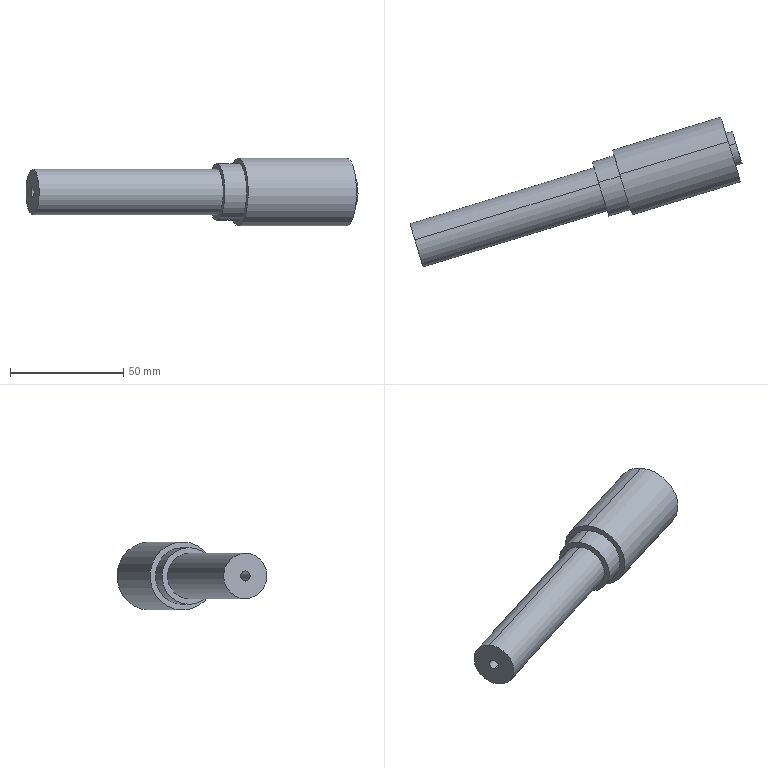Component | SolidWorks | V1ZHXTRotatingAxisSB1-1 | 1 solid | 34 faces | box 146.66 x 66.23 x 30 mm | volume 66443 mm3 | cylinder 20 | cone 8 | plane 6 | commonest cylinder face diameters 3.3 x6 4 x2 4.496 x2 15 x2 2 x2 30 x2 25 x2 20 x2
build123d program:
from build123d import *

# Parameters (mm, degrees)
SKETCH1_R                  = 10
BOSS_EXTRUDE1_DEPTH        = 85
SKETCH2_R                  = 12.5
BOSS_EXTRUDE2_DEPTH        = 10
SKETCH3_R                  = 15
BOSS_EXTRUDE3_DEPTH        = 50
SKETCH4_R                  = 1
CUT_EXTRUDE1_DEPTH         = 147.544
BOSS_EXTRUDE4_START        = 3
SKETCH5_R                  = 7.5
SKETCH5_R_2                = 1
BOSS_EXTRUDE4_DEPTH        = 3
M4_TAPPED_HOLE1_D          = 3.3
M4_TAPPED_HOLE1_DEPTH      = 10.1
M4_TAPPED_HOLE1_TIP        = 0.9914
F_12_24_TAPPED_HOLE1_D     = 4.496
F_12_24_TAPPED_HOLE1_DEPTH = 14.15
F_12_24_TAPPED_HOLE1_TIP   = 1.351
SKETCH10_R                 = 2
CUT_EXTRUDE2_DEPTH         = 10


with BuildPart() as part:
    # Sketch1 → Boss-Extrude1 (new body)
    with BuildSketch(Plane(origin=(0, 0, 0), x_dir=(1, 0, 0), z_dir=(0, 1, 0))):
        with Locations(Location((0, 0, 0), (0, 0, 270))):
            Circle(SKETCH1_R)
    extrude(amount=BOSS_EXTRUDE1_DEPTH)

    # Sketch2 → Boss-Extrude2 (add)
    with BuildSketch(Plane(origin=(0, 85, 0), x_dir=(1, 0, 0), z_dir=(0, 1, 0))):
        with Locations(Location((0, 0, 0), (0, 0, 270))):
            Circle(SKETCH2_R)
    extrude(amount=BOSS_EXTRUDE2_DEPTH)

    # Sketch3 → Boss-Extrude3 (add)
    with BuildSketch(Plane(origin=(0, 95, 0), x_dir=(1, 0, 0), z_dir=(0, 1, 0))):
        with Locations(Location((0, 0, 0), (0, 0, 270))):
            Circle(SKETCH3_R)
    extrude(amount=BOSS_EXTRUDE3_DEPTH)

    # Sketch4 → Cut-Extrude1 (cut, through all)
    with BuildSketch(Plane(origin=(0, 145, 0), x_dir=(1, 0, 0), z_dir=(0, 1, 0))):
        with Locations(Location((0, 0, 0), (0, 0, 270))):
            Circle(SKETCH4_R)
    extrude(amount=-CUT_EXTRUDE1_DEPTH, mode=Mode.SUBTRACT)

    # Sketch5 → Boss-Extrude4 (add)
    with BuildSketch(Plane(origin=(0, 145, 0), x_dir=(1, 0, 0), z_dir=(0, 1, 0)).offset(BOSS_EXTRUDE4_START)):
        with Locations(Location((0, 0, 0), (0, 0, 270))):
            Circle(SKETCH5_R)
        with Locations(Location((0, 0, 0), (0, 0, 270))):
            Circle(SKETCH5_R_2, mode=Mode.SUBTRACT)
    extrude(amount=-BOSS_EXTRUDE4_DEPTH)

    # M4 Tapped Hole1
    with Locations(Plane(origin=(0, 145, 0), x_dir=(1, 0, 0), z_dir=(0, 1, 0))):
        with Locations((0, 11), (-9.526, -5.5), (9.526, -5.5)):
            Hole(M4_TAPPED_HOLE1_D / 2, depth=M4_TAPPED_HOLE1_DEPTH)
            with Locations((0, 0, -(M4_TAPPED_HOLE1_DEPTH + M4_TAPPED_HOLE1_TIP / 2))):  # 118° drill point
                Cone(0, M4_TAPPED_HOLE1_D / 2, M4_TAPPED_HOLE1_TIP, mode=Mode.SUBTRACT)

    # 12-24 Tapped Hole1
    with Locations(Plane(origin=(0, 0, 0), x_dir=(-1, 0, 0), z_dir=(0, -1, 0))):
        with Locations((0, 0)):
            Hole(F_12_24_TAPPED_HOLE1_D / 2, depth=F_12_24_TAPPED_HOLE1_DEPTH)
            with Locations((0, 0, -(F_12_24_TAPPED_HOLE1_DEPTH + F_12_24_TAPPED_HOLE1_TIP / 2))):  # 118° drill point
                Cone(0, F_12_24_TAPPED_HOLE1_D / 2, F_12_24_TAPPED_HOLE1_TIP, mode=Mode.SUBTRACT)

    # Sketch10 → Cut-Extrude2 (cut)
    with BuildSketch(Plane(origin=(0, 145, 0), x_dir=(1, 0, 0), z_dir=(0, 1, 0))):
        with Locations(Location((9.526, 5.5, 0), (0, 0, 270))):
            Circle(SKETCH10_R)
    extrude(amount=-CUT_EXTRUDE2_DEPTH, mode=Mode.SUBTRACT)


solid = part.part

# Placed as in the assembly
solid = solid.moved(Location((147.067, -241.347, 375.239), (-13.538, -4.085, -73.517)))
STEP:
#1=COLOUR_RGB('',0.7922,0.8196,0.9333);
#2=FILL_AREA_STYLE_COLOUR('',#1);
#3=FILL_AREA_STYLE('',(#2));
#4=SURFACE_STYLE_FILL_AREA(#3);
#5=SURFACE_SIDE_STYLE('',(#4));
#6=SURFACE_STYLE_USAGE(.BOTH.,#5);
#7=PRESENTATION_STYLE_ASSIGNMENT((#6));
#8=CARTESIAN_POINT('',(11.001,-8.368,14.578));
#9=VERTEX_POINT('',#8);
#10=CARTESIAN_POINT('',(10.99,-8.331,14.731));
#11=VERTEX_POINT('',#10);
#12=CARTESIAN_POINT('',(10.995,-8.349,14.655));
#13=DIRECTION('',(0.9565,0.2918,0.));
#14=DIRECTION('',(-0.07124,0.2335,0.9697));
#15=AXIS2_PLACEMENT_3D('',#12,#13,#14);
#16=CIRCLE('',#15,0.07874);
#17=EDGE_CURVE('',#9,#11,#16,.T.);
#18=ORIENTED_EDGE('',*,*,#17,.F.);
#19=CARTESIAN_POINT('',(11.377,-8.253,14.578));
#20=VERTEX_POINT('',#19);
#21=CARTESIAN_POINT('',(11.001,-8.368,14.578));
#22=DIRECTION('',(0.9565,0.2918,0.));
#23=VECTOR('',#22,39.37);
#24=LINE('',#21,#23);
#25=EDGE_CURVE('',#9,#20,#24,.T.);
#26=ORIENTED_EDGE('',*,*,#25,.T.);
#27=CARTESIAN_POINT('',(11.366,-8.216,14.731));
#28=VERTEX_POINT('',#27);
#29=CARTESIAN_POINT('',(11.372,-8.234,14.655));
#30=DIRECTION('',(0.9565,0.2918,0.));
#31=DIRECTION('',(-0.07124,0.2335,0.9697));
#32=AXIS2_PLACEMENT_3D('',#29,#30,#31);
#33=CIRCLE('',#32,0.07874);
#34=EDGE_CURVE('',#20,#28,#33,.T.);
#35=ORIENTED_EDGE('',*,*,#34,.T.);
#36=CARTESIAN_POINT('',(10.99,-8.331,14.731));
#37=DIRECTION('',(0.9565,0.2918,0.));
#38=VECTOR('',#37,39.37);
#39=LINE('',#36,#38);
#40=EDGE_CURVE('',#11,#28,#39,.T.);
#41=ORIENTED_EDGE('',*,*,#40,.F.);
#42=EDGE_LOOP('',(#18,#26,#35,#41));
#43=FACE_OUTER_BOUND('',#42,.T.);
#44=CARTESIAN_POINT('',(10.995,-8.349,14.655));
#45=DIRECTION('',(0.9565,0.2918,0.));
#46=DIRECTION('',(-0.07124,0.2335,0.9697));
#47=AXIS2_PLACEMENT_3D('',#44,#45,#46);
#48=CYLINDRICAL_SURFACE('',#47,0.07874);
#49=ADVANCED_FACE('',(#43),#48,.F.);
#50=CARTESIAN_POINT('',(6.317,-9.319,14.859));
#51=VERTEX_POINT('',#50);
#52=CARTESIAN_POINT('',(6.329,-9.36,14.687));
#53=VERTEX_POINT('',#52);
#54=CARTESIAN_POINT('',(6.323,-9.339,14.773));
#55=DIRECTION('',(-0.9565,-0.2918,-0.));
#56=DIRECTION('',(0.07124,-0.2335,-0.9697));
#57=AXIS2_PLACEMENT_3D('',#54,#55,#56);
#58=CIRCLE('',#57,0.0885);
#59=EDGE_CURVE('',#51,#53,#58,.T.);
#60=ORIENTED_EDGE('',*,*,#59,.F.);
#61=CARTESIAN_POINT('',(5.784,-9.481,14.859));
#62=VERTEX_POINT('',#61);
#63=CARTESIAN_POINT('',(5.784,-9.481,14.859));
#64=DIRECTION('',(-0.9565,-0.2918,-0.));
#65=VECTOR('',#64,39.37);
#66=LINE('',#63,#65);
#67=EDGE_CURVE('',#51,#62,#66,.T.);
#68=ORIENTED_EDGE('',*,*,#67,.T.);
#69=CARTESIAN_POINT('',(5.796,-9.523,14.687));
#70=VERTEX_POINT('',#69);
#71=CARTESIAN_POINT('',(5.79,-9.502,14.773));
#72=DIRECTION('',(-0.9565,-0.2918,-0.));
#73=DIRECTION('',(0.07124,-0.2335,-0.9697));
#74=AXIS2_PLACEMENT_3D('',#71,#72,#73);
#75=CIRCLE('',#74,0.0885);
#76=EDGE_CURVE('',#62,#70,#75,.T.);
#77=ORIENTED_EDGE('',*,*,#76,.T.);
#78=CARTESIAN_POINT('',(5.796,-9.523,14.687));
#79=DIRECTION('',(-0.9565,-0.2918,-0.));
#80=VECTOR('',#79,39.37);
#81=LINE('',#78,#80);
#82=EDGE_CURVE('',#53,#70,#81,.T.);
#83=ORIENTED_EDGE('',*,*,#82,.F.);
#84=EDGE_LOOP('',(#60,#68,#77,#83));
#85=FACE_OUTER_BOUND('',#84,.T.);
#86=CARTESIAN_POINT('',(5.79,-9.502,14.773));
#87=DIRECTION('',(-0.9565,-0.2918,-0.));
#88=DIRECTION('',(0.07124,-0.2335,-0.9697));
#89=AXIS2_PLACEMENT_3D('',#86,#87,#88);
#90=CYLINDRICAL_SURFACE('',#89,0.0885);
#91=ADVANCED_FACE('',(#85),#90,.F.);
#92=CARTESIAN_POINT('',(6.348,-9.321,14.811));
#93=VERTEX_POINT('',#92);
#94=CARTESIAN_POINT('',(6.354,-9.34,14.735));
#95=VERTEX_POINT('',#94);
#96=CARTESIAN_POINT('',(6.351,-9.331,14.773));
#97=DIRECTION('',(-0.9565,-0.2918,-0.));
#98=DIRECTION('',(0.07124,-0.2335,-0.9697));
#99=AXIS2_PLACEMENT_3D('',#96,#97,#98);
#100=CIRCLE('',#99,0.03937);
#101=EDGE_CURVE('',#93,#95,#100,.T.);
#102=ORIENTED_EDGE('',*,*,#101,.F.);
#103=CARTESIAN_POINT('',(6.317,-9.319,14.859));
#104=DIRECTION('',(-0.5537,0.04984,0.8312));
#105=VECTOR('',#104,39.37);
#106=LINE('',#103,#105);
#107=EDGE_CURVE('',#93,#51,#106,.T.);
#108=ORIENTED_EDGE('',*,*,#107,.T.);
#109=ORIENTED_EDGE('',*,*,#59,.T.);
#110=CARTESIAN_POINT('',(6.329,-9.36,14.687));
#111=DIRECTION('',(-0.4316,-0.3504,-0.8312));
#112=VECTOR('',#111,39.37);
#113=LINE('',#110,#112);
#114=EDGE_CURVE('',#95,#53,#113,.T.);
#115=ORIENTED_EDGE('',*,*,#114,.F.);
#116=EDGE_LOOP('',(#102,#108,#109,#115));
#117=FACE_OUTER_BOUND('',#116,.T.);
#118=CARTESIAN_POINT('',(6.323,-9.339,14.773));
#119=DIRECTION('',(-0.9565,-0.2918,-0.));
#120=DIRECTION('',(0.07124,-0.2335,-0.9697));
#121=AXIS2_PLACEMENT_3D('',#118,#119,#120);
#122=CONICAL_SURFACE('',#121,0.0885,1.03);
#123=ADVANCED_FACE('',(#117),#122,.F.);
#124=CARTESIAN_POINT('',(10.905,-8.068,14.29));
#125=VERTEX_POINT('',#124);
#126=CARTESIAN_POINT('',(10.896,-8.038,14.416));
#127=VERTEX_POINT('',#126);
#128=CARTESIAN_POINT('',(10.901,-8.053,14.353));
#129=DIRECTION('',(0.9565,0.2918,0.));
#130=DIRECTION('',(-0.07124,0.2335,0.9697));
#131=AXIS2_PLACEMENT_3D('',#128,#129,#130);
#132=CIRCLE('',#131,0.06496);
#133=EDGE_CURVE('',#125,#127,#132,.T.);
#134=ORIENTED_EDGE('',*,*,#133,.F.);
#135=CARTESIAN_POINT('',(11.286,-7.952,14.29));
#136=VERTEX_POINT('',#135);
#137=CARTESIAN_POINT('',(11.286,-7.952,14.29));
#138=DIRECTION('',(0.9565,0.2918,0.));
#139=VECTOR('',#138,39.37);
#140=LINE('',#137,#139);
#141=EDGE_CURVE('',#125,#136,#140,.T.);
#142=ORIENTED_EDGE('',*,*,#141,.T.);
#143=CARTESIAN_POINT('',(11.276,-7.922,14.416));
#144=VERTEX_POINT('',#143);
#145=CARTESIAN_POINT('',(11.281,-7.937,14.353));
#146=DIRECTION('',(0.9565,0.2918,0.));
#147=DIRECTION('',(-0.07124,0.2335,0.9697));
#148=AXIS2_PLACEMENT_3D('',#145,#146,#147);
#149=CIRCLE('',#148,0.06496);
#150=EDGE_CURVE('',#136,#144,#149,.T.);
#151=ORIENTED_EDGE('',*,*,#150,.T.);
#152=CARTESIAN_POINT('',(11.276,-7.922,14.416));
#153=DIRECTION('',(0.9565,0.2918,0.));
#154=VECTOR('',#153,39.37);
#155=LINE('',#152,#154);
#156=EDGE_CURVE('',#127,#144,#155,.T.);
#157=ORIENTED_EDGE('',*,*,#156,.F.);
#158=EDGE_LOOP('',(#134,#142,#151,#157));
#159=FACE_OUTER_BOUND('',#158,.T.);
#160=CARTESIAN_POINT('',(11.281,-7.937,14.353));
#161=DIRECTION('',(0.9565,0.2918,0.));
#162=DIRECTION('',(-0.07124,0.2335,0.9697));
#163=AXIS2_PLACEMENT_3D('',#160,#161,#162);
#164=CYLINDRICAL_SURFACE('',#163,0.06496);
#165=ADVANCED_FACE('',(#159),#164,.F.);
#166=CARTESIAN_POINT('',(10.863,-8.064,14.353));
#167=VERTEX_POINT('',#166);
#168=CARTESIAN_POINT('',(10.896,-8.038,14.416));
#169=DIRECTION('',(0.4316,0.3504,0.8312));
#170=VECTOR('',#169,39.37);
#171=LINE('',#168,#170);
#172=EDGE_CURVE('',#167,#127,#171,.T.);
#173=ORIENTED_EDGE('',*,*,#172,.F.);
#174=CARTESIAN_POINT('',(10.905,-8.068,14.29));
#175=DIRECTION('',(0.5537,-0.04984,-0.8312));
#176=VECTOR('',#175,39.37);
#177=LINE('',#174,#176);
#178=EDGE_CURVE('',#167,#125,#177,.T.);
#179=ORIENTED_EDGE('',*,*,#178,.T.);
#180=ORIENTED_EDGE('',*,*,#133,.T.);
#181=EDGE_LOOP('',(#173,#179,#180));
#182=FACE_OUTER_BOUND('',#181,.T.);
#183=CARTESIAN_POINT('',(10.901,-8.053,14.353));
#184=DIRECTION('',(0.9565,0.2918,0.));
#185=DIRECTION('',(-0.07124,0.2335,0.9697));
#186=AXIS2_PLACEMENT_3D('',#183,#184,#185);
#187=CONICAL_SURFACE('',#186,0.06496,1.03);
#188=ADVANCED_FACE('',(#182),#187,.F.);
#189=CARTESIAN_POINT('',(10.753,-7.569,14.829));
#190=VERTEX_POINT('',#189);
#191=CARTESIAN_POINT('',(10.744,-7.538,14.955));
#192=VERTEX_POINT('',#191);
#193=CARTESIAN_POINT('',(10.748,-7.554,14.892));
#194=DIRECTION('',(0.9565,0.2918,0.));
#195=DIRECTION('',(-0.07124,0.2335,0.9697));
#196=AXIS2_PLACEMENT_3D('',#193,#194,#195);
#197=CIRCLE('',#196,0.06496);
#198=EDGE_CURVE('',#190,#192,#197,.T.);
#199=ORIENTED_EDGE('',*,*,#198,.F.);
#200=CARTESIAN_POINT('',(11.133,-7.453,14.829));
#201=VERTEX_POINT('',#200);
#202=CARTESIAN_POINT('',(11.133,-7.453,14.829));
#203=DIRECTION('',(0.9565,0.2918,0.));
#204=VECTOR('',#203,39.37);
#205=LINE('',#202,#204);
#206=EDGE_CURVE('',#190,#201,#205,.T.);
#207=ORIENTED_EDGE('',*,*,#206,.T.);
#208=CARTESIAN_POINT('',(11.124,-7.422,14.955));
#209=VERTEX_POINT('',#208);
#210=CARTESIAN_POINT('',(11.129,-7.437,14.892));
#211=DIRECTION('',(0.9565,0.2918,0.));
#212=DIRECTION('',(-0.07124,0.2335,0.9697));
#213=AXIS2_PLACEMENT_3D('',#210,#211,#212);
#214=CIRCLE('',#213,0.06496);
#215=EDGE_CURVE('',#201,#209,#214,.T.);
#216=ORIENTED_EDGE('',*,*,#215,.T.);
#217=CARTESIAN_POINT('',(11.124,-7.422,14.955));
#218=DIRECTION('',(0.9565,0.2918,0.));
#219=VECTOR('',#218,39.37);
#220=LINE('',#217,#219);
#221=EDGE_CURVE('',#192,#209,#220,.T.);
#222=ORIENTED_EDGE('',*,*,#221,.F.);
#223=EDGE_LOOP('',(#199,#207,#216,#222));
#224=FACE_OUTER_BOUND('',#223,.T.);
#225=CARTESIAN_POINT('',(11.129,-7.437,14.892));
#226=DIRECTION('',(0.9565,0.2918,0.));
#227=DIRECTION('',(-0.07124,0.2335,0.9697));
#228=AXIS2_PLACEMENT_3D('',#225,#226,#227);
#229=CYLINDRICAL_SURFACE('',#228,0.06496);
#230=ADVANCED_FACE('',(#224),#229,.F.);
#231=CARTESIAN_POINT('',(10.711,-7.565,14.892));
#232=VERTEX_POINT('',#231);
#233=CARTESIAN_POINT('',(10.744,-7.538,14.955));
#234=DIRECTION('',(0.4316,0.3504,0.8312));
#235=VECTOR('',#234,39.37);
#236=LINE('',#233,#235);
#237=EDGE_CURVE('',#232,#192,#236,.T.);
#238=ORIENTED_EDGE('',*,*,#237,.F.);
#239=CARTESIAN_POINT('',(10.753,-7.569,14.829));
#240=DIRECTION('',(0.5537,-0.04984,-0.8312));
#241=VECTOR('',#240,39.37);
#242=LINE('',#239,#241);
#243=EDGE_CURVE('',#232,#190,#242,.T.);
#244=ORIENTED_EDGE('',*,*,#243,.T.);
#245=ORIENTED_EDGE('',*,*,#198,.T.);
#246=EDGE_LOOP('',(#238,#244,#245));
#247=FACE_OUTER_BOUND('',#246,.T.);
#248=CARTESIAN_POINT('',(10.748,-7.554,14.892));
#249=DIRECTION('',(0.9565,0.2918,0.));
#250=DIRECTION('',(-0.07124,0.2335,0.9697));
#251=AXIS2_PLACEMENT_3D('',#248,#249,#250);
#252=CONICAL_SURFACE('',#251,0.06496,1.03);
#253=ADVANCED_FACE('',(#247),#252,.F.);
#254=CARTESIAN_POINT('',(10.965,-8.264,15.012));
#255=VERTEX_POINT('',#254);
#256=CARTESIAN_POINT('',(10.956,-8.234,15.138));
#257=VERTEX_POINT('',#256);
#258=CARTESIAN_POINT('',(10.961,-8.249,15.075));
#259=DIRECTION('',(0.9565,0.2918,0.));
#260=DIRECTION('',(-0.07124,0.2335,0.9697));
#261=AXIS2_PLACEMENT_3D('',#258,#259,#260);
#262=CIRCLE('',#261,0.06496);
#263=EDGE_CURVE('',#255,#257,#262,.T.);
#264=ORIENTED_EDGE('',*,*,#263,.F.);
#265=CARTESIAN_POINT('',(11.346,-8.148,15.012));
#266=VERTEX_POINT('',#265);
#267=CARTESIAN_POINT('',(11.346,-8.148,15.012));
#268=DIRECTION('',(0.9565,0.2918,0.));
#269=VECTOR('',#268,39.37);
#270=LINE('',#267,#269);
#271=EDGE_CURVE('',#255,#266,#270,.T.);
#272=ORIENTED_EDGE('',*,*,#271,.T.);
#273=CARTESIAN_POINT('',(11.336,-8.118,15.138));
#274=VERTEX_POINT('',#273);
#275=CARTESIAN_POINT('',(11.341,-8.133,15.075));
#276=DIRECTION('',(0.9565,0.2918,0.));
#277=DIRECTION('',(-0.07124,0.2335,0.9697));
#278=AXIS2_PLACEMENT_3D('',#275,#276,#277);
#279=CIRCLE('',#278,0.06496);
#280=EDGE_CURVE('',#266,#274,#279,.T.);
#281=ORIENTED_EDGE('',*,*,#280,.T.);
#282=CARTESIAN_POINT('',(11.336,-8.118,15.138));
#283=DIRECTION('',(0.9565,0.2918,0.));
#284=VECTOR('',#283,39.37);
#285=LINE('',#282,#284);
#286=EDGE_CURVE('',#257,#274,#285,.T.);
#287=ORIENTED_EDGE('',*,*,#286,.F.);
#288=EDGE_LOOP('',(#264,#272,#281,#287));
#289=FACE_OUTER_BOUND('',#288,.T.);
#290=CARTESIAN_POINT('',(11.341,-8.133,15.075));
#291=DIRECTION('',(0.9565,0.2918,0.));
#292=DIRECTION('',(-0.07124,0.2335,0.9697));
#293=AXIS2_PLACEMENT_3D('',#290,#291,#292);
#294=CYLINDRICAL_SURFACE('',#293,0.06496);
#295=ADVANCED_FACE('',(#289),#294,.F.);
#296=CARTESIAN_POINT('',(10.923,-8.261,15.075));
#297=VERTEX_POINT('',#296);
#298=CARTESIAN_POINT('',(10.956,-8.234,15.138));
#299=DIRECTION('',(0.4316,0.3504,0.8312));
#300=VECTOR('',#299,39.37);
#301=LINE('',#298,#300);
#302=EDGE_CURVE('',#297,#257,#301,.T.);
#303=ORIENTED_EDGE('',*,*,#302,.F.);
#304=CARTESIAN_POINT('',(10.965,-8.264,15.012));
#305=DIRECTION('',(0.5537,-0.04984,-0.8312));
#306=VECTOR('',#305,39.37);
#307=LINE('',#304,#306);
#308=EDGE_CURVE('',#297,#255,#307,.T.);
#309=ORIENTED_EDGE('',*,*,#308,.T.);
#310=ORIENTED_EDGE('',*,*,#263,.T.);
#311=EDGE_LOOP('',(#303,#309,#310));
#312=FACE_OUTER_BOUND('',#311,.T.);
#313=CARTESIAN_POINT('',(10.961,-8.249,15.075));
#314=DIRECTION('',(0.9565,0.2918,0.));
#315=DIRECTION('',(-0.07124,0.2335,0.9697));
#316=AXIS2_PLACEMENT_3D('',#313,#314,#315);
#317=CONICAL_SURFACE('',#316,0.06496,1.03);
#318=ADVANCED_FACE('',(#312),#317,.F.);
#319=CARTESIAN_POINT('',(11.342,-7.732,15.06));
#320=VERTEX_POINT('',#319);
#321=CARTESIAN_POINT('',(11.384,-7.87,14.487));
#322=VERTEX_POINT('',#321);
#323=CARTESIAN_POINT('',(11.363,-7.801,14.773));
#324=DIRECTION('',(0.9565,0.2918,0.));
#325=DIRECTION('',(-0.07124,0.2335,0.9697));
#326=AXIS2_PLACEMENT_3D('',#323,#324,#325);
#327=CIRCLE('',#326,0.2953);
#328=EDGE_CURVE('',#320,#322,#327,.T.);
#329=ORIENTED_EDGE('',*,*,#328,.F.);
#330=CARTESIAN_POINT('',(11.229,-7.767,15.06));
#331=VERTEX_POINT('',#330);
#332=CARTESIAN_POINT('',(11.342,-7.732,15.06));
#333=DIRECTION('',(-0.9565,-0.2918,-0.));
#334=VECTOR('',#333,39.37);
#335=LINE('',#332,#334);
#336=EDGE_CURVE('',#320,#331,#335,.T.);
#337=ORIENTED_EDGE('',*,*,#336,.T.);
#338=CARTESIAN_POINT('',(11.271,-7.905,14.487));
#339=VERTEX_POINT('',#338);
#340=CARTESIAN_POINT('',(11.25,-7.836,14.773));
#341=DIRECTION('',(0.9565,0.2918,0.));
#342=DIRECTION('',(-0.07124,0.2335,0.9697));
#343=AXIS2_PLACEMENT_3D('',#340,#341,#342);
#344=CIRCLE('',#343,0.2953);
#345=EDGE_CURVE('',#331,#339,#344,.T.);
#346=ORIENTED_EDGE('',*,*,#345,.T.);
#347=CARTESIAN_POINT('',(11.384,-7.87,14.487));
#348=DIRECTION('',(-0.9565,-0.2918,-0.));
#349=VECTOR('',#348,39.37);
#350=LINE('',#347,#349);
#351=EDGE_CURVE('',#322,#339,#350,.T.);
#352=ORIENTED_EDGE('',*,*,#351,.F.);
#353=EDGE_LOOP('',(#329,#337,#346,#352));
#354=FACE_OUTER_BOUND('',#353,.T.);
#355=CARTESIAN_POINT('',(11.363,-7.801,14.773));
#356=DIRECTION('',(-0.9565,-0.2918,-0.));
#357=DIRECTION('',(0.07124,-0.2335,-0.9697));
#358=AXIS2_PLACEMENT_3D('',#355,#356,#357);
#359=CYLINDRICAL_SURFACE('',#358,0.2953);
#360=ADVANCED_FACE('',(#354),#359,.T.);
#361=ORIENTED_EDGE('',*,*,#101,.T.);
#362=CARTESIAN_POINT('',(11.366,-7.811,14.735));
#363=VERTEX_POINT('',#362);
#364=CARTESIAN_POINT('',(5.793,-9.511,14.735));
#365=DIRECTION('',(0.9565,0.2918,0.));
#366=VECTOR('',#365,39.37);
#367=LINE('',#364,#366);
#368=EDGE_CURVE('',#95,#363,#367,.T.);
#369=ORIENTED_EDGE('',*,*,#368,.T.);
#370=CARTESIAN_POINT('',(11.36,-7.792,14.811));
#371=VERTEX_POINT('',#370);
#372=CARTESIAN_POINT('',(11.363,-7.801,14.773));
#373=DIRECTION('',(0.9565,0.2918,0.));
#374=DIRECTION('',(-0.07124,0.2335,0.9697));
#375=AXIS2_PLACEMENT_3D('',#372,#373,#374);
#376=CIRCLE('',#375,0.03937);
#377=EDGE_CURVE('',#363,#371,#376,.T.);
#378=ORIENTED_EDGE('',*,*,#377,.T.);
#379=CARTESIAN_POINT('',(5.787,-9.493,14.811));
#380=DIRECTION('',(0.9565,0.2918,0.));
#381=VECTOR('',#380,39.37);
#382=LINE('',#379,#381);
#383=EDGE_CURVE('',#93,#371,#382,.T.);
#384=ORIENTED_EDGE('',*,*,#383,.F.);
#385=EDGE_LOOP('',(#361,#369,#378,#384));
#386=FACE_OUTER_BOUND('',#385,.T.);
#387=CARTESIAN_POINT('',(5.79,-9.502,14.773));
#388=DIRECTION('',(0.9565,0.2918,0.));
#389=DIRECTION('',(-0.07124,0.2335,0.9697));
#390=AXIS2_PLACEMENT_3D('',#387,#388,#389);
#391=CYLINDRICAL_SURFACE('',#390,0.03937);
#392=ADVANCED_FACE('',(#386),#391,.F.);
#393=CARTESIAN_POINT('',(11.208,-7.698,15.346));
#394=VERTEX_POINT('',#393);
#395=CARTESIAN_POINT('',(11.292,-7.974,14.201));
#396=VERTEX_POINT('',#395);
#397=CARTESIAN_POINT('',(11.25,-7.836,14.773));
#398=DIRECTION('',(0.9565,0.2918,0.));
#399=DIRECTION('',(-0.07124,0.2335,0.9697));
#400=AXIS2_PLACEMENT_3D('',#397,#398,#399);
#401=CIRCLE('',#400,0.5906);
#402=EDGE_CURVE('',#394,#396,#401,.T.);
#403=ORIENTED_EDGE('',*,*,#402,.F.);
#404=CARTESIAN_POINT('',(9.325,-8.272,15.346));
#405=VERTEX_POINT('',#404);
#406=CARTESIAN_POINT('',(11.208,-7.698,15.346));
#407=DIRECTION('',(-0.9565,-0.2918,-0.));
#408=VECTOR('',#407,39.37);
#409=LINE('',#406,#408);
#410=EDGE_CURVE('',#394,#405,#409,.T.);
#411=ORIENTED_EDGE('',*,*,#410,.T.);
#412=CARTESIAN_POINT('',(9.409,-8.548,14.201));
#413=VERTEX_POINT('',#412);
#414=CARTESIAN_POINT('',(9.367,-8.41,14.773));
#415=DIRECTION('',(0.9565,0.2918,0.));
#416=DIRECTION('',(-0.07124,0.2335,0.9697));
#417=AXIS2_PLACEMENT_3D('',#414,#415,#416);
#418=CIRCLE('',#417,0.5906);
#419=EDGE_CURVE('',#405,#413,#418,.T.);
#420=ORIENTED_EDGE('',*,*,#419,.T.);
#421=CARTESIAN_POINT('',(11.292,-7.974,14.201));
#422=DIRECTION('',(-0.9565,-0.2918,-0.));
#423=VECTOR('',#422,39.37);
#424=LINE('',#421,#423);
#425=EDGE_CURVE('',#396,#413,#424,.T.);
#426=ORIENTED_EDGE('',*,*,#425,.F.);
#427=EDGE_LOOP('',(#403,#411,#420,#426));
#428=FACE_OUTER_BOUND('',#427,.T.);
#429=CARTESIAN_POINT('',(11.25,-7.836,14.773));
#430=DIRECTION('',(-0.9565,-0.2918,-0.));
#431=DIRECTION('',(0.07124,-0.2335,-0.9697));
#432=AXIS2_PLACEMENT_3D('',#429,#430,#431);
#433=CYLINDRICAL_SURFACE('',#432,0.5906);
#434=ADVANCED_FACE('',(#428),#433,.T.);
#435=CARTESIAN_POINT('',(9.332,-8.295,15.25));
#436=VERTEX_POINT('',#435);
#437=CARTESIAN_POINT('',(9.402,-8.525,14.296));
#438=VERTEX_POINT('',#437);
#439=CARTESIAN_POINT('',(9.367,-8.41,14.773));
#440=DIRECTION('',(0.9565,0.2918,0.));
#441=DIRECTION('',(-0.07124,0.2335,0.9697));
#442=AXIS2_PLACEMENT_3D('',#439,#440,#441);
#443=CIRCLE('',#442,0.4921);
#444=EDGE_CURVE('',#436,#438,#443,.T.);
#445=ORIENTED_EDGE('',*,*,#444,.F.);
#446=CARTESIAN_POINT('',(8.956,-8.41,15.25));
#447=VERTEX_POINT('',#446);
#448=CARTESIAN_POINT('',(9.332,-8.295,15.25));
#449=DIRECTION('',(-0.9565,-0.2918,-0.));
#450=VECTOR('',#449,39.37);
#451=LINE('',#448,#450);
#452=EDGE_CURVE('',#436,#447,#451,.T.);
#453=ORIENTED_EDGE('',*,*,#452,.T.);
#454=CARTESIAN_POINT('',(9.026,-8.64,14.296));
#455=VERTEX_POINT('',#454);
#456=CARTESIAN_POINT('',(8.991,-8.525,14.773));
#457=DIRECTION('',(0.9565,0.2918,0.));
#458=DIRECTION('',(-0.07124,0.2335,0.9697));
#459=AXIS2_PLACEMENT_3D('',#456,#457,#458);
#460=CIRCLE('',#459,0.4921);
#461=EDGE_CURVE('',#447,#455,#460,.T.);
#462=ORIENTED_EDGE('',*,*,#461,.T.);
#463=CARTESIAN_POINT('',(9.402,-8.525,14.296));
#464=DIRECTION('',(-0.9565,-0.2918,-0.));
#465=VECTOR('',#464,39.37);
#466=LINE('',#463,#465);
#467=EDGE_CURVE('',#438,#455,#466,.T.);
#468=ORIENTED_EDGE('',*,*,#467,.F.);
#469=EDGE_LOOP('',(#445,#453,#462,#468));
#470=FACE_OUTER_BOUND('',#469,.T.);
#471=CARTESIAN_POINT('',(9.367,-8.41,14.773));
#472=DIRECTION('',(-0.9565,-0.2918,-0.));
#473=DIRECTION('',(0.07124,-0.2335,-0.9697));
#474=AXIS2_PLACEMENT_3D('',#471,#472,#473);
#475=CYLINDRICAL_SURFACE('',#474,0.4921);
#476=ADVANCED_FACE('',(#470),#475,.T.);
#477=CARTESIAN_POINT('',(8.963,-8.433,15.155));
#478=VERTEX_POINT('',#477);
#479=CARTESIAN_POINT('',(9.019,-8.617,14.391));
#480=VERTEX_POINT('',#479);
#481=CARTESIAN_POINT('',(8.991,-8.525,14.773));
#482=DIRECTION('',(0.9565,0.2918,0.));
#483=DIRECTION('',(-0.07124,0.2335,0.9697));
#484=AXIS2_PLACEMENT_3D('',#481,#482,#483);
#485=CIRCLE('',#484,0.3937);
#486=EDGE_CURVE('',#478,#480,#485,.T.);
#487=ORIENTED_EDGE('',*,*,#486,.F.);
#488=CARTESIAN_POINT('',(5.762,-9.41,15.155));
#489=VERTEX_POINT('',#488);
#490=CARTESIAN_POINT('',(8.963,-8.433,15.155));
#491=DIRECTION('',(-0.9565,-0.2918,-0.));
#492=VECTOR('',#491,39.37);
#493=LINE('',#490,#492);
#494=EDGE_CURVE('',#478,#489,#493,.T.);
#495=ORIENTED_EDGE('',*,*,#494,.T.);
#496=CARTESIAN_POINT('',(5.818,-9.594,14.391));
#497=VERTEX_POINT('',#496);
#498=CARTESIAN_POINT('',(5.79,-9.502,14.773));
#499=DIRECTION('',(0.9565,0.2918,0.));
#500=DIRECTION('',(-0.07124,0.2335,0.9697));
#501=AXIS2_PLACEMENT_3D('',#498,#499,#500);
#502=CIRCLE('',#501,0.3937);
#503=EDGE_CURVE('',#489,#497,#502,.T.);
#504=ORIENTED_EDGE('',*,*,#503,.T.);
#505=CARTESIAN_POINT('',(9.019,-8.617,14.391));
#506=DIRECTION('',(-0.9565,-0.2918,-0.));
#507=VECTOR('',#506,39.37);
#508=LINE('',#505,#507);
#509=EDGE_CURVE('',#480,#497,#508,.T.);
#510=ORIENTED_EDGE('',*,*,#509,.F.);
#511=EDGE_LOOP('',(#487,#495,#504,#510));
#512=FACE_OUTER_BOUND('',#511,.T.);
#513=CARTESIAN_POINT('',(8.991,-8.525,14.773));
#514=DIRECTION('',(-0.9565,-0.2918,-0.));
#515=DIRECTION('',(0.07124,-0.2335,-0.9697));
#516=AXIS2_PLACEMENT_3D('',#513,#514,#515);
#517=CYLINDRICAL_SURFACE('',#516,0.3937);
#518=ADVANCED_FACE('',(#512),#517,.T.);
#519=CARTESIAN_POINT('',(11.372,-8.234,14.655));
#520=DIRECTION('',(0.9565,0.2918,0.));
#521=DIRECTION('',(-0.07124,0.2335,0.9697));
#522=AXIS2_PLACEMENT_3D('',#519,#520,#521);
#523=CIRCLE('',#522,0.07874);
#524=EDGE_CURVE('',#28,#20,#523,.T.);
#525=ORIENTED_EDGE('',*,*,#524,.F.);
#526=ORIENTED_EDGE('',*,*,#34,.F.);
#527=EDGE_LOOP('',(#525,#526));
#528=FACE_BOUND('',#527,.T.);
#529=CARTESIAN_POINT('',(11.281,-7.937,14.353));
#530=DIRECTION('',(0.9565,0.2918,0.));
#531=DIRECTION('',(-0.07124,0.2335,0.9697));
#532=AXIS2_PLACEMENT_3D('',#529,#530,#531);
#533=CIRCLE('',#532,0.06496);
#534=EDGE_CURVE('',#144,#136,#533,.T.);
#535=ORIENTED_EDGE('',*,*,#534,.F.);
#536=ORIENTED_EDGE('',*,*,#150,.F.);
#537=EDGE_LOOP('',(#535,#536));
#538=FACE_BOUND('',#537,.T.);
#539=CARTESIAN_POINT('',(11.129,-7.437,14.892));
#540=DIRECTION('',(0.9565,0.2918,0.));
#541=DIRECTION('',(-0.07124,0.2335,0.9697));
#542=AXIS2_PLACEMENT_3D('',#539,#540,#541);
#543=CIRCLE('',#542,0.06496);
#544=EDGE_CURVE('',#209,#201,#543,.T.);
#545=ORIENTED_EDGE('',*,*,#544,.F.);
#546=ORIENTED_EDGE('',*,*,#215,.F.);
#547=EDGE_LOOP('',(#545,#546));
#548=FACE_BOUND('',#547,.T.);
#549=CARTESIAN_POINT('',(11.341,-8.133,15.075));
#550=DIRECTION('',(0.9565,0.2918,0.));
#551=DIRECTION('',(-0.07124,0.2335,0.9697));
#552=AXIS2_PLACEMENT_3D('',#549,#550,#551);
#553=CIRCLE('',#552,0.06496);
#554=EDGE_CURVE('',#274,#266,#553,.T.);
#555=ORIENTED_EDGE('',*,*,#554,.F.);
#556=ORIENTED_EDGE('',*,*,#280,.F.);
#557=EDGE_LOOP('',(#555,#556));
#558=FACE_BOUND('',#557,.T.);
#559=CARTESIAN_POINT('',(11.25,-7.836,14.773));
#560=DIRECTION('',(0.9565,0.2918,0.));
#561=DIRECTION('',(-0.07124,0.2335,0.9697));
#562=AXIS2_PLACEMENT_3D('',#559,#560,#561);
#563=CIRCLE('',#562,0.5906);
#564=EDGE_CURVE('',#396,#394,#563,.T.);
#565=ORIENTED_EDGE('',*,*,#564,.T.);
#566=ORIENTED_EDGE('',*,*,#402,.T.);
#567=EDGE_LOOP('',(#565,#566));
#568=FACE_OUTER_BOUND('',#567,.T.);
#569=CARTESIAN_POINT('',(11.25,-7.836,14.773));
#570=DIRECTION('',(0.9565,0.2918,0.));
#571=DIRECTION('',(-0.07124,0.2335,0.9697));
#572=AXIS2_PLACEMENT_3D('',#569,#570,#571);
#573=CIRCLE('',#572,0.2953);
#574=EDGE_CURVE('',#339,#331,#573,.T.);
#575=ORIENTED_EDGE('',*,*,#574,.F.);
#576=ORIENTED_EDGE('',*,*,#345,.F.);
#577=EDGE_LOOP('',(#575,#576));
#578=FACE_BOUND('',#577,.T.);
#579=CARTESIAN_POINT('',(11.25,-7.836,14.773));
#580=DIRECTION('',(0.9565,0.2918,0.));
#581=DIRECTION('',(-0.07124,0.2335,0.9697));
#582=AXIS2_PLACEMENT_3D('',#579,#580,#581);
#583=PLANE('',#582);
#584=ADVANCED_FACE('',(#528,#538,#548,#558,#568,#578),#583,.T.);
#585=ORIENTED_EDGE('',*,*,#494,.F.);
#586=CARTESIAN_POINT('',(8.991,-8.525,14.773));
#587=DIRECTION('',(0.9565,0.2918,0.));
#588=DIRECTION('',(-0.07124,0.2335,0.9697));
#589=AXIS2_PLACEMENT_3D('',#586,#587,#588);
#590=CIRCLE('',#589,0.3937);
#591=EDGE_CURVE('',#480,#478,#590,.T.);
#592=ORIENTED_EDGE('',*,*,#591,.F.);
#593=ORIENTED_EDGE('',*,*,#509,.T.);
#594=CARTESIAN_POINT('',(5.79,-9.502,14.773));
#595=DIRECTION('',(0.9565,0.2918,0.));
#596=DIRECTION('',(-0.07124,0.2335,0.9697));
#597=AXIS2_PLACEMENT_3D('',#594,#595,#596);
#598=CIRCLE('',#597,0.3937);
#599=EDGE_CURVE('',#497,#489,#598,.T.);
#600=ORIENTED_EDGE('',*,*,#599,.T.);
#601=EDGE_LOOP('',(#585,#592,#593,#600));
#602=FACE_OUTER_BOUND('',#601,.T.);
#603=CARTESIAN_POINT('',(8.991,-8.525,14.773));
#604=DIRECTION('',(-0.9565,-0.2918,-0.));
#605=DIRECTION('',(0.07124,-0.2335,-0.9697));
#606=AXIS2_PLACEMENT_3D('',#603,#604,#605);
#607=CYLINDRICAL_SURFACE('',#606,0.3937);
#608=ADVANCED_FACE('',(#602),#607,.T.);
#609=CARTESIAN_POINT('',(5.79,-9.502,14.773));
#610=DIRECTION('',(-0.9565,-0.2918,-0.));
#611=DIRECTION('',(0.07124,-0.2335,-0.9697));
#612=AXIS2_PLACEMENT_3D('',#609,#610,#611);
#613=CIRCLE('',#612,0.0885);
#614=EDGE_CURVE('',#70,#62,#613,.T.);
#615=ORIENTED_EDGE('',*,*,#614,.F.);
#616=ORIENTED_EDGE('',*,*,#76,.F.);
#617=EDGE_LOOP('',(#615,#616));
#618=FACE_BOUND('',#617,.T.);
#619=ORIENTED_EDGE('',*,*,#599,.F.);
#620=ORIENTED_EDGE('',*,*,#503,.F.);
#621=EDGE_LOOP('',(#619,#620));
#622=FACE_OUTER_BOUND('',#621,.T.);
#623=CARTESIAN_POINT('',(5.79,-9.502,14.773));
#624=DIRECTION('',(0.9565,0.2918,0.));
#625=DIRECTION('',(-0.07124,0.2335,0.9697));
#626=AXIS2_PLACEMENT_3D('',#623,#624,#625);
#627=PLANE('',#626);
#628=ADVANCED_FACE('',(#618,#622),#627,.F.);
#629=ORIENTED_EDGE('',*,*,#452,.F.);
#630=CARTESIAN_POINT('',(9.367,-8.41,14.773));
#631=DIRECTION('',(0.9565,0.2918,0.));
#632=DIRECTION('',(-0.07124,0.2335,0.9697));
#633=AXIS2_PLACEMENT_3D('',#630,#631,#632);
#634=CIRCLE('',#633,0.4921);
#635=EDGE_CURVE('',#438,#436,#634,.T.);
#636=ORIENTED_EDGE('',*,*,#635,.F.);
#637=ORIENTED_EDGE('',*,*,#467,.T.);
#638=CARTESIAN_POINT('',(8.991,-8.525,14.773));
#639=DIRECTION('',(0.9565,0.2918,0.));
#640=DIRECTION('',(-0.07124,0.2335,0.9697));
#641=AXIS2_PLACEMENT_3D('',#638,#639,#640);
#642=CIRCLE('',#641,0.4921);
#643=EDGE_CURVE('',#455,#447,#642,.T.);
#644=ORIENTED_EDGE('',*,*,#643,.T.);
#645=EDGE_LOOP('',(#629,#636,#637,#644));
#646=FACE_OUTER_BOUND('',#645,.T.);
#647=CARTESIAN_POINT('',(9.367,-8.41,14.773));
#648=DIRECTION('',(-0.9565,-0.2918,-0.));
#649=DIRECTION('',(0.07124,-0.2335,-0.9697));
#650=AXIS2_PLACEMENT_3D('',#647,#648,#649);
#651=CYLINDRICAL_SURFACE('',#650,0.4921);
#652=ADVANCED_FACE('',(#646),#651,.T.);
#653=ORIENTED_EDGE('',*,*,#591,.T.);
#654=ORIENTED_EDGE('',*,*,#486,.T.);
#655=EDGE_LOOP('',(#653,#654));
#656=FACE_BOUND('',#655,.T.);
#657=ORIENTED_EDGE('',*,*,#643,.F.);
#658=ORIENTED_EDGE('',*,*,#461,.F.);
#659=EDGE_LOOP('',(#657,#658));
#660=FACE_OUTER_BOUND('',#659,.T.);
#661=CARTESIAN_POINT('',(8.991,-8.525,14.773));
#662=DIRECTION('',(0.9565,0.2918,0.));
#663=DIRECTION('',(-0.07124,0.2335,0.9697));
#664=AXIS2_PLACEMENT_3D('',#661,#662,#663);
#665=PLANE('',#664);
#666=ADVANCED_FACE('',(#656,#660),#665,.F.);
#667=ORIENTED_EDGE('',*,*,#410,.F.);
#668=ORIENTED_EDGE('',*,*,#564,.F.);
#669=ORIENTED_EDGE('',*,*,#425,.T.);
#670=CARTESIAN_POINT('',(9.367,-8.41,14.773));
#671=DIRECTION('',(0.9565,0.2918,0.));
#672=DIRECTION('',(-0.07124,0.2335,0.9697));
#673=AXIS2_PLACEMENT_3D('',#670,#671,#672);
#674=CIRCLE('',#673,0.5906);
#675=EDGE_CURVE('',#413,#405,#674,.T.);
#676=ORIENTED_EDGE('',*,*,#675,.T.);
#677=EDGE_LOOP('',(#667,#668,#669,#676));
#678=FACE_OUTER_BOUND('',#677,.T.);
#679=CARTESIAN_POINT('',(11.25,-7.836,14.773));
#680=DIRECTION('',(-0.9565,-0.2918,-0.));
#681=DIRECTION('',(0.07124,-0.2335,-0.9697));
#682=AXIS2_PLACEMENT_3D('',#679,#680,#681);
#683=CYLINDRICAL_SURFACE('',#682,0.5906);
#684=ADVANCED_FACE('',(#678),#683,.T.);
#685=ORIENTED_EDGE('',*,*,#635,.T.);
#686=ORIENTED_EDGE('',*,*,#444,.T.);
#687=EDGE_LOOP('',(#685,#686));
#688=FACE_BOUND('',#687,.T.);
#689=ORIENTED_EDGE('',*,*,#675,.F.);
#690=ORIENTED_EDGE('',*,*,#419,.F.);
#691=EDGE_LOOP('',(#689,#690));
#692=FACE_OUTER_BOUND('',#691,.T.);
#693=CARTESIAN_POINT('',(9.367,-8.41,14.773));
#694=DIRECTION('',(0.9565,0.2918,0.));
#695=DIRECTION('',(-0.07124,0.2335,0.9697));
#696=AXIS2_PLACEMENT_3D('',#693,#694,#695);
#697=PLANE('',#696);
#698=ADVANCED_FACE('',(#688,#692),#697,.F.);
#699=ORIENTED_EDGE('',*,*,#368,.F.);
#700=CARTESIAN_POINT('',(6.351,-9.331,14.773));
#701=DIRECTION('',(-0.9565,-0.2918,-0.));
#702=DIRECTION('',(0.07124,-0.2335,-0.9697));
#703=AXIS2_PLACEMENT_3D('',#700,#701,#702);
#704=CIRCLE('',#703,0.03937);
#705=EDGE_CURVE('',#95,#93,#704,.T.);
#706=ORIENTED_EDGE('',*,*,#705,.T.);
#707=ORIENTED_EDGE('',*,*,#383,.T.);
#708=CARTESIAN_POINT('',(11.363,-7.801,14.773));
#709=DIRECTION('',(0.9565,0.2918,0.));
#710=DIRECTION('',(-0.07124,0.2335,0.9697));
#711=AXIS2_PLACEMENT_3D('',#708,#709,#710);
#712=CIRCLE('',#711,0.03937);
#713=EDGE_CURVE('',#371,#363,#712,.T.);
#714=ORIENTED_EDGE('',*,*,#713,.T.);
#715=EDGE_LOOP('',(#699,#706,#707,#714));
#716=FACE_OUTER_BOUND('',#715,.T.);
#717=CARTESIAN_POINT('',(5.79,-9.502,14.773));
#718=DIRECTION('',(0.9565,0.2918,0.));
#719=DIRECTION('',(-0.07124,0.2335,0.9697));
#720=AXIS2_PLACEMENT_3D('',#717,#718,#719);
#721=CYLINDRICAL_SURFACE('',#720,0.03937);
#722=ADVANCED_FACE('',(#716),#721,.F.);
#723=CARTESIAN_POINT('',(11.363,-7.801,14.773));
#724=DIRECTION('',(0.9565,0.2918,0.));
#725=DIRECTION('',(-0.07124,0.2335,0.9697));
#726=AXIS2_PLACEMENT_3D('',#723,#724,#725);
#727=CIRCLE('',#726,0.2953);
#728=EDGE_CURVE('',#322,#320,#727,.T.);
#729=ORIENTED_EDGE('',*,*,#728,.T.);
#730=ORIENTED_EDGE('',*,*,#328,.T.);
#731=EDGE_LOOP('',(#729,#730));
#732=FACE_OUTER_BOUND('',#731,.T.);
#733=ORIENTED_EDGE('',*,*,#713,.F.);
#734=ORIENTED_EDGE('',*,*,#377,.F.);
#735=EDGE_LOOP('',(#733,#734));
#736=FACE_BOUND('',#735,.T.);
#737=CARTESIAN_POINT('',(11.363,-7.801,14.773));
#738=DIRECTION('',(0.9565,0.2918,0.));
#739=DIRECTION('',(-0.07124,0.2335,0.9697));
#740=AXIS2_PLACEMENT_3D('',#737,#738,#739);
#741=PLANE('',#740);
#742=ADVANCED_FACE('',(#732,#736),#741,.T.);
#743=ORIENTED_EDGE('',*,*,#336,.F.);
#744=ORIENTED_EDGE('',*,*,#728,.F.);
#745=ORIENTED_EDGE('',*,*,#351,.T.);
#746=ORIENTED_EDGE('',*,*,#574,.T.);
#747=EDGE_LOOP('',(#743,#744,#745,#746));
#748=FACE_OUTER_BOUND('',#747,.T.);
#749=CARTESIAN_POINT('',(11.363,-7.801,14.773));
#750=DIRECTION('',(-0.9565,-0.2918,-0.));
#751=DIRECTION('',(0.07124,-0.2335,-0.9697));
#752=AXIS2_PLACEMENT_3D('',#749,#750,#751);
#753=CYLINDRICAL_SURFACE('',#752,0.2953);
#754=ADVANCED_FACE('',(#748),#753,.T.);
#755=ORIENTED_EDGE('',*,*,#308,.F.);
#756=ORIENTED_EDGE('',*,*,#302,.T.);
#757=CARTESIAN_POINT('',(10.961,-8.249,15.075));
#758=DIRECTION('',(0.9565,0.2918,0.));
#759=DIRECTION('',(-0.07124,0.2335,0.9697));
#760=AXIS2_PLACEMENT_3D('',#757,#758,#759);
#761=CIRCLE('',#760,0.06496);
#762=EDGE_CURVE('',#257,#255,#761,.T.);
#763=ORIENTED_EDGE('',*,*,#762,.T.);
#764=EDGE_LOOP('',(#755,#756,#763));
#765=FACE_OUTER_BOUND('',#764,.T.);
#766=CARTESIAN_POINT('',(10.961,-8.249,15.075));
#767=DIRECTION('',(0.9565,0.2918,0.));
#768=DIRECTION('',(-0.07124,0.2335,0.9697));
#769=AXIS2_PLACEMENT_3D('',#766,#767,#768);
#770=CONICAL_SURFACE('',#769,0.06496,1.03);
#771=ADVANCED_FACE('',(#765),#770,.F.);
#772=ORIENTED_EDGE('',*,*,#271,.F.);
#773=ORIENTED_EDGE('',*,*,#762,.F.);
#774=ORIENTED_EDGE('',*,*,#286,.T.);
#775=ORIENTED_EDGE('',*,*,#554,.T.);
#776=EDGE_LOOP('',(#772,#773,#774,#775));
#777=FACE_OUTER_BOUND('',#776,.T.);
#778=CARTESIAN_POINT('',(11.341,-8.133,15.075));
#779=DIRECTION('',(0.9565,0.2918,0.));
#780=DIRECTION('',(-0.07124,0.2335,0.9697));
#781=AXIS2_PLACEMENT_3D('',#778,#779,#780);
#782=CYLINDRICAL_SURFACE('',#781,0.06496);
#783=ADVANCED_FACE('',(#777),#782,.F.);
#784=ORIENTED_EDGE('',*,*,#243,.F.);
#785=ORIENTED_EDGE('',*,*,#237,.T.);
#786=CARTESIAN_POINT('',(10.748,-7.554,14.892));
#787=DIRECTION('',(0.9565,0.2918,0.));
#788=DIRECTION('',(-0.07124,0.2335,0.9697));
#789=AXIS2_PLACEMENT_3D('',#786,#787,#788);
#790=CIRCLE('',#789,0.06496);
#791=EDGE_CURVE('',#192,#190,#790,.T.);
#792=ORIENTED_EDGE('',*,*,#791,.T.);
#793=EDGE_LOOP('',(#784,#785,#792));
#794=FACE_OUTER_BOUND('',#793,.T.);
#795=CARTESIAN_POINT('',(10.748,-7.554,14.892));
#796=DIRECTION('',(0.9565,0.2918,0.));
#797=DIRECTION('',(-0.07124,0.2335,0.9697));
#798=AXIS2_PLACEMENT_3D('',#795,#796,#797);
#799=CONICAL_SURFACE('',#798,0.06496,1.03);
#800=ADVANCED_FACE('',(#794),#799,.F.);
#801=ORIENTED_EDGE('',*,*,#206,.F.);
#802=ORIENTED_EDGE('',*,*,#791,.F.);
#803=ORIENTED_EDGE('',*,*,#221,.T.);
#804=ORIENTED_EDGE('',*,*,#544,.T.);
#805=EDGE_LOOP('',(#801,#802,#803,#804));
#806=FACE_OUTER_BOUND('',#805,.T.);
#807=CARTESIAN_POINT('',(11.129,-7.437,14.892));
#808=DIRECTION('',(0.9565,0.2918,0.));
#809=DIRECTION('',(-0.07124,0.2335,0.9697));
#810=AXIS2_PLACEMENT_3D('',#807,#808,#809);
#811=CYLINDRICAL_SURFACE('',#810,0.06496);
#812=ADVANCED_FACE('',(#806),#811,.F.);
#813=ORIENTED_EDGE('',*,*,#178,.F.);
#814=ORIENTED_EDGE('',*,*,#172,.T.);
#815=CARTESIAN_POINT('',(10.901,-8.053,14.353));
#816=DIRECTION('',(0.9565,0.2918,0.));
#817=DIRECTION('',(-0.07124,0.2335,0.9697));
#818=AXIS2_PLACEMENT_3D('',#815,#816,#817);
#819=CIRCLE('',#818,0.06496);
#820=EDGE_CURVE('',#127,#125,#819,.T.);
#821=ORIENTED_EDGE('',*,*,#820,.T.);
#822=EDGE_LOOP('',(#813,#814,#821));
#823=FACE_OUTER_BOUND('',#822,.T.);
#824=CARTESIAN_POINT('',(10.901,-8.053,14.353));
#825=DIRECTION('',(0.9565,0.2918,0.));
#826=DIRECTION('',(-0.07124,0.2335,0.9697));
#827=AXIS2_PLACEMENT_3D('',#824,#825,#826);
#828=CONICAL_SURFACE('',#827,0.06496,1.03);
#829=ADVANCED_FACE('',(#823),#828,.F.);
#830=ORIENTED_EDGE('',*,*,#141,.F.);
#831=ORIENTED_EDGE('',*,*,#820,.F.);
#832=ORIENTED_EDGE('',*,*,#156,.T.);
#833=ORIENTED_EDGE('',*,*,#534,.T.);
#834=EDGE_LOOP('',(#830,#831,#832,#833));
#835=FACE_OUTER_BOUND('',#834,.T.);
#836=CARTESIAN_POINT('',(11.281,-7.937,14.353));
#837=DIRECTION('',(0.9565,0.2918,0.));
#838=DIRECTION('',(-0.07124,0.2335,0.9697));
#839=AXIS2_PLACEMENT_3D('',#836,#837,#838);
#840=CYLINDRICAL_SURFACE('',#839,0.06496);
#841=ADVANCED_FACE('',(#835),#840,.F.);
#842=ORIENTED_EDGE('',*,*,#107,.F.);
#843=ORIENTED_EDGE('',*,*,#705,.F.);
#844=ORIENTED_EDGE('',*,*,#114,.T.);
#845=CARTESIAN_POINT('',(6.323,-9.339,14.773));
#846=DIRECTION('',(-0.9565,-0.2918,-0.));
#847=DIRECTION('',(0.07124,-0.2335,-0.9697));
#848=AXIS2_PLACEMENT_3D('',#845,#846,#847);
#849=CIRCLE('',#848,0.0885);
#850=EDGE_CURVE('',#53,#51,#849,.T.);
#851=ORIENTED_EDGE('',*,*,#850,.T.);
#852=EDGE_LOOP('',(#842,#843,#844,#851));
#853=FACE_OUTER_BOUND('',#852,.T.);
#854=CARTESIAN_POINT('',(6.323,-9.339,14.773));
#855=DIRECTION('',(-0.9565,-0.2918,-0.));
#856=DIRECTION('',(0.07124,-0.2335,-0.9697));
#857=AXIS2_PLACEMENT_3D('',#854,#855,#856);
#858=CONICAL_SURFACE('',#857,0.0885,1.03);
#859=ADVANCED_FACE('',(#853),#858,.F.);
#860=ORIENTED_EDGE('',*,*,#67,.F.);
#861=ORIENTED_EDGE('',*,*,#850,.F.);
#862=ORIENTED_EDGE('',*,*,#82,.T.);
#863=ORIENTED_EDGE('',*,*,#614,.T.);
#864=EDGE_LOOP('',(#860,#861,#862,#863));
#865=FACE_OUTER_BOUND('',#864,.T.);
#866=CARTESIAN_POINT('',(5.79,-9.502,14.773));
#867=DIRECTION('',(-0.9565,-0.2918,-0.));
#868=DIRECTION('',(0.07124,-0.2335,-0.9697));
#869=AXIS2_PLACEMENT_3D('',#866,#867,#868);
#870=CYLINDRICAL_SURFACE('',#869,0.0885);
#871=ADVANCED_FACE('',(#865),#870,.F.);
#872=ORIENTED_EDGE('',*,*,#25,.F.);
#873=CARTESIAN_POINT('',(10.995,-8.349,14.655));
#874=DIRECTION('',(0.9565,0.2918,0.));
#875=DIRECTION('',(-0.07124,0.2335,0.9697));
#876=AXIS2_PLACEMENT_3D('',#873,#874,#875);
#877=CIRCLE('',#876,0.07874);
#878=EDGE_CURVE('',#11,#9,#877,.T.);
#879=ORIENTED_EDGE('',*,*,#878,.F.);
#880=ORIENTED_EDGE('',*,*,#40,.T.);
#881=ORIENTED_EDGE('',*,*,#524,.T.);
#882=EDGE_LOOP('',(#872,#879,#880,#881));
#883=FACE_OUTER_BOUND('',#882,.T.);
#884=CARTESIAN_POINT('',(10.995,-8.349,14.655));
#885=DIRECTION('',(0.9565,0.2918,0.));
#886=DIRECTION('',(-0.07124,0.2335,0.9697));
#887=AXIS2_PLACEMENT_3D('',#884,#885,#886);
#888=CYLINDRICAL_SURFACE('',#887,0.07874);
#889=ADVANCED_FACE('',(#883),#888,.F.);
#890=ORIENTED_EDGE('',*,*,#878,.T.);
#891=ORIENTED_EDGE('',*,*,#17,.T.);
#892=EDGE_LOOP('',(#890,#891));
#893=FACE_OUTER_BOUND('',#892,.T.);
#894=CARTESIAN_POINT('',(10.995,-8.349,14.655));
#895=DIRECTION('',(0.9565,0.2918,0.));
#896=DIRECTION('',(-0.07124,0.2335,0.9697));
#897=AXIS2_PLACEMENT_3D('',#894,#895,#896);
#898=PLANE('',#897);
#899=ADVANCED_FACE('',(#893),#898,.T.);
#900=CLOSED_SHELL('',(#49,#91,#123,#165,#188,#230,#253,#295,#318,#360,#392,#434,#476,#518,#584,#608,#628,#652,#666,#684,#698,#722,#742,#754,#771,#783,#800,#812,#829,#841,#859,#871,#889,#899));
#901=MANIFOLD_SOLID_BREP('',#900);
#902=STYLED_ITEM('',(#7),#901);
#903=PRESENTATION_LAYER_ASSIGNMENT('','',(#902));
#904=CARTESIAN_POINT('',(0.,0.,0.));
#905=DIRECTION('',(0.,0.,1.));
#906=DIRECTION('',(1.,0.,0.));
#907=AXIS2_PLACEMENT_3D('',#904,#905,#906);
#908=(LENGTH_UNIT()NAMED_UNIT(*)SI_UNIT($,.METRE.));
#909=LENGTH_MEASURE_WITH_UNIT(LENGTH_MEASURE(0.0254),#908);
#910=DIMENSIONAL_EXPONENTS(1.,0.,0.,0.,0.,0.,0.);
#911=(CONVERSION_BASED_UNIT('',#909)LENGTH_UNIT()NAMED_UNIT(#910));
#912=UNCERTAINTY_MEASURE_WITH_UNIT(LENGTH_MEASURE(0.00001),#911,'','');
#913=(NAMED_UNIT(*)PLANE_ANGLE_UNIT()SI_UNIT($,.RADIAN.));
#914=(NAMED_UNIT(*)SI_UNIT($,.STERADIAN.)SOLID_ANGLE_UNIT());
#915=(GEOMETRIC_REPRESENTATION_CONTEXT(3)GLOBAL_UNCERTAINTY_ASSIGNED_CONTEXT((#912))GLOBAL_UNIT_ASSIGNED_CONTEXT((#911,#913,#914))REPRESENTATION_CONTEXT('',''));
#916=ADVANCED_BREP_SHAPE_REPRESENTATION('',(#901,#907),#915);
#917=(LENGTH_UNIT()NAMED_UNIT(*)SI_UNIT($,.METRE.));
#918=LENGTH_MEASURE_WITH_UNIT(LENGTH_MEASURE(0.0254),#917);
#919=DIMENSIONAL_EXPONENTS(1.,0.,0.,0.,0.,0.,0.);
#920=(CONVERSION_BASED_UNIT('',#918)LENGTH_UNIT()NAMED_UNIT(#919));
#921=UNCERTAINTY_MEASURE_WITH_UNIT(LENGTH_MEASURE(0.00001),#920,'','');
#922=(NAMED_UNIT(*)PLANE_ANGLE_UNIT()SI_UNIT($,.RADIAN.));
#923=(NAMED_UNIT(*)SI_UNIT($,.STERADIAN.)SOLID_ANGLE_UNIT());
#924=(GEOMETRIC_REPRESENTATION_CONTEXT(3)GLOBAL_UNCERTAINTY_ASSIGNED_CONTEXT((#921))GLOBAL_UNIT_ASSIGNED_CONTEXT((#920,#922,#923))REPRESENTATION_CONTEXT('',''));
#925=MECHANICAL_DESIGN_GEOMETRIC_PRESENTATION_REPRESENTATION('',(#902),#924);